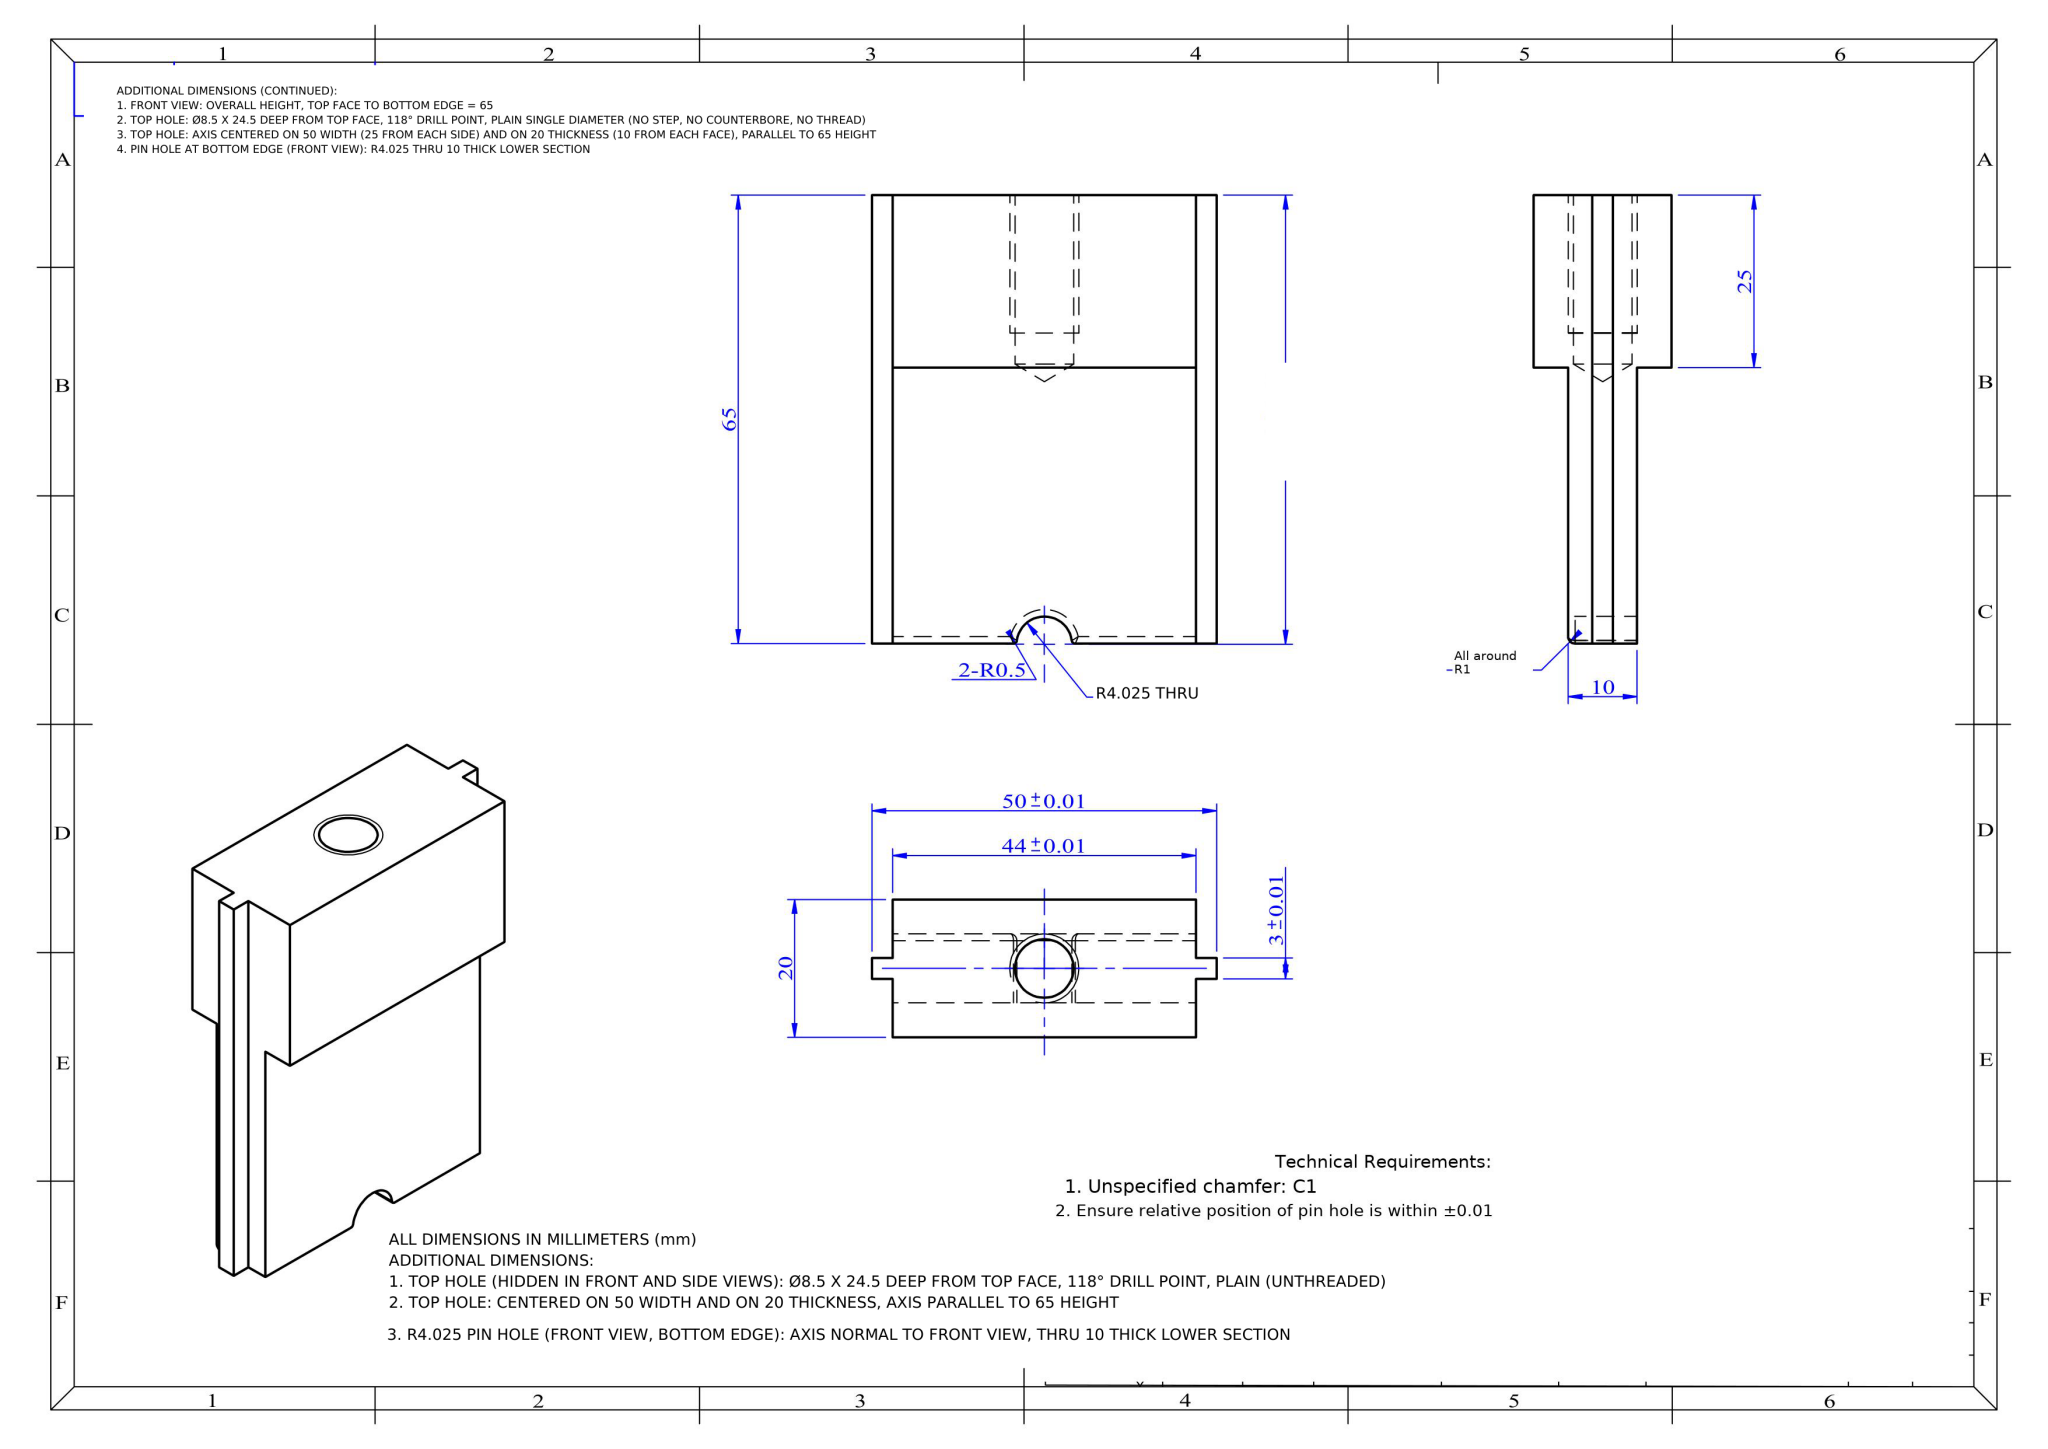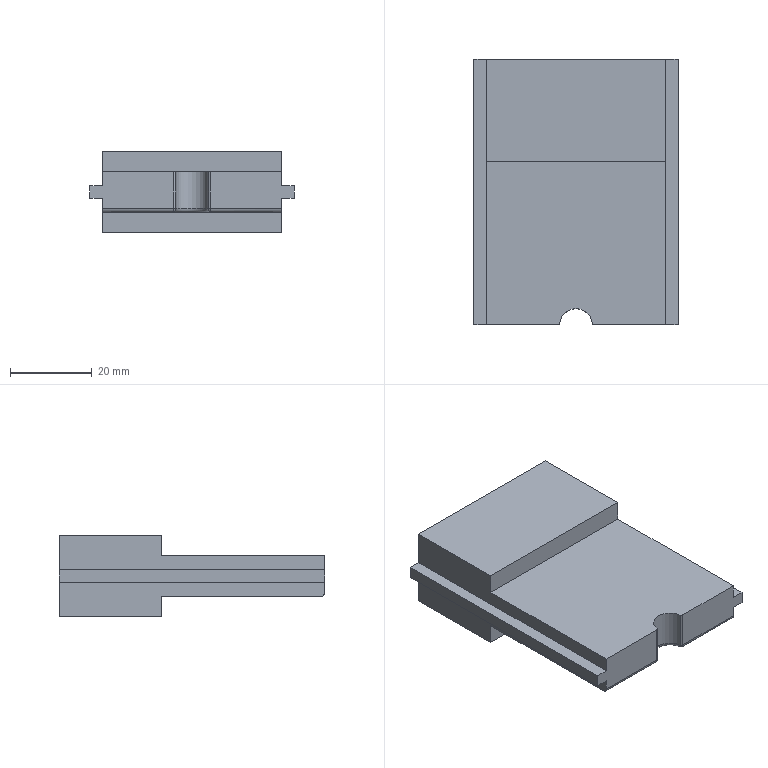Part | NX | mm | 1 solid | 31 faces | box 50 x 65 x 20 mm | volume 39074 mm3 | plane 19 | cylinder 7 | cone 2 | spline 2 | torus 1 | commonest cylinder face diameters 8.5 x2 1 x2 2 x2 8.05 x1